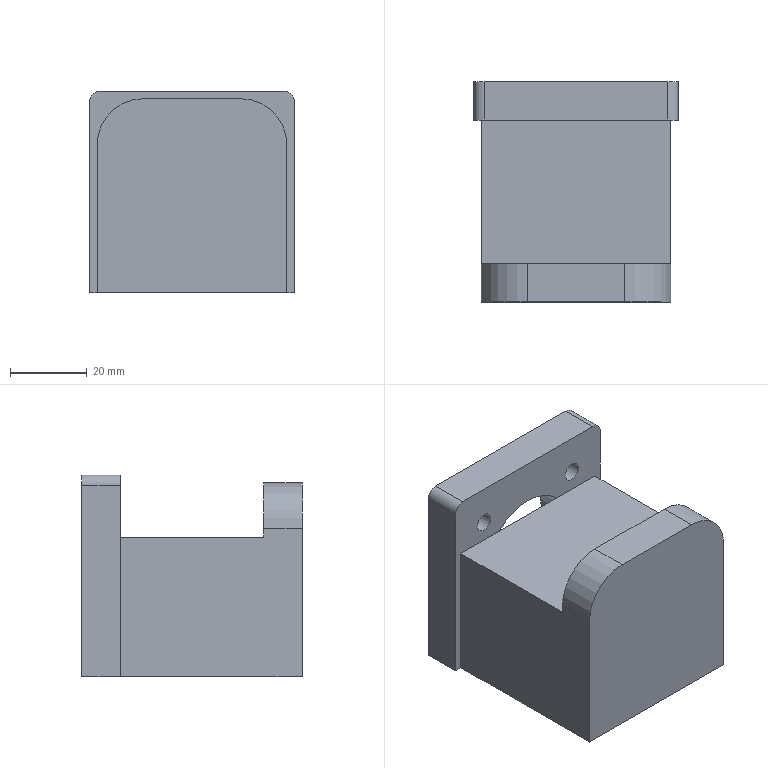Component | SolidWorks | 3359524133GTH5-400-BC(2)-1__GTH5.-BC_body6^3359524133GTH5-400-BC(2)-1 | 1 solid | 29 faces | box 53.5 x 57.5 x 52.7 mm | volume 112565 mm3 | plane 15 | cylinder 14 | commonest cylinder face diameters 4.917 x8 30 x2 24 x2 5.5 x2
STEP:
#1=COLOUR_RGB('',0.7922,0.8196,0.9333);
#2=FILL_AREA_STYLE_COLOUR('',#1);
#3=FILL_AREA_STYLE('',(#2));
#4=SURFACE_STYLE_FILL_AREA(#3);
#5=SURFACE_SIDE_STYLE('',(#4));
#6=SURFACE_STYLE_USAGE(.BOTH.,#5);
#7=PRESENTATION_STYLE_ASSIGNMENT((#6));
#8=CARTESIAN_POINT('',(13.795,57.972,-86.659));
#9=VERTEX_POINT('',#8);
#10=CARTESIAN_POINT('',(13.626,57.972,-87.072));
#11=VERTEX_POINT('',#10);
#12=CARTESIAN_POINT('',(14.216,57.972,-87.072));
#13=DIRECTION('',(0.,-1.,-0.));
#14=DIRECTION('',(1.,0.,0.));
#15=AXIS2_PLACEMENT_3D('',#12,#13,#14);
#16=CIRCLE('',#15,0.5906);
#17=EDGE_CURVE('',#9,#11,#16,.T.);
#18=ORIENTED_EDGE('',*,*,#17,.T.);
#19=CARTESIAN_POINT('',(13.626,58.366,-87.072));
#20=VERTEX_POINT('',#19);
#21=CARTESIAN_POINT('',(13.626,57.972,-87.072));
#22=DIRECTION('',(0.,1.,0.));
#23=VECTOR('',#22,39.37);
#24=LINE('',#21,#23);
#25=EDGE_CURVE('',#11,#20,#24,.T.);
#26=ORIENTED_EDGE('',*,*,#25,.T.);
#27=CARTESIAN_POINT('',(14.807,58.366,-87.072));
#28=VERTEX_POINT('',#27);
#29=CARTESIAN_POINT('',(14.216,58.366,-87.072));
#30=DIRECTION('',(0.,-1.,-0.));
#31=DIRECTION('',(1.,0.,0.));
#32=AXIS2_PLACEMENT_3D('',#29,#30,#31);
#33=CIRCLE('',#32,0.5906);
#34=EDGE_CURVE('',#28,#20,#33,.T.);
#35=ORIENTED_EDGE('',*,*,#34,.F.);
#36=CARTESIAN_POINT('',(14.807,57.972,-87.072));
#37=VERTEX_POINT('',#36);
#38=CARTESIAN_POINT('',(14.807,57.972,-87.072));
#39=DIRECTION('',(0.,1.,0.));
#40=VECTOR('',#39,39.37);
#41=LINE('',#38,#40);
#42=EDGE_CURVE('',#37,#28,#41,.T.);
#43=ORIENTED_EDGE('',*,*,#42,.F.);
#44=CARTESIAN_POINT('',(14.638,57.972,-86.659));
#45=VERTEX_POINT('',#44);
#46=CARTESIAN_POINT('',(14.216,57.972,-87.072));
#47=DIRECTION('',(0.,-1.,-0.));
#48=DIRECTION('',(1.,0.,0.));
#49=AXIS2_PLACEMENT_3D('',#46,#47,#48);
#50=CIRCLE('',#49,0.5906);
#51=EDGE_CURVE('',#37,#45,#50,.T.);
#52=ORIENTED_EDGE('',*,*,#51,.T.);
#53=CARTESIAN_POINT('',(14.216,57.972,-87.072));
#54=DIRECTION('',(0.,-1.,-0.));
#55=DIRECTION('',(1.,0.,0.));
#56=AXIS2_PLACEMENT_3D('',#53,#54,#55);
#57=CIRCLE('',#56,0.5906);
#58=EDGE_CURVE('',#45,#9,#57,.T.);
#59=ORIENTED_EDGE('',*,*,#58,.T.);
#60=EDGE_LOOP('',(#18,#26,#35,#43,#52,#59));
#61=FACE_OUTER_BOUND('',#60,.T.);
#62=CARTESIAN_POINT('',(14.216,57.972,-87.072));
#63=DIRECTION('',(0.,1.,0.));
#64=DIRECTION('',(1.,0.,0.));
#65=AXIS2_PLACEMENT_3D('',#62,#63,#64);
#66=CYLINDRICAL_SURFACE('',#65,0.5906);
#67=ADVANCED_FACE('',(#61),#66,.F.);
#68=CARTESIAN_POINT('',(13.673,57.972,-87.714));
#69=VERTEX_POINT('',#68);
#70=CARTESIAN_POINT('',(13.48,57.972,-87.714));
#71=VERTEX_POINT('',#70);
#72=CARTESIAN_POINT('',(13.577,57.972,-87.714));
#73=DIRECTION('',(0.,-1.,-0.));
#74=DIRECTION('',(1.,0.,0.));
#75=AXIS2_PLACEMENT_3D('',#72,#73,#74);
#76=CIRCLE('',#75,0.09679);
#77=EDGE_CURVE('',#69,#71,#76,.T.);
#78=ORIENTED_EDGE('',*,*,#77,.T.);
#79=CARTESIAN_POINT('',(13.48,58.366,-87.714));
#80=VERTEX_POINT('',#79);
#81=CARTESIAN_POINT('',(13.48,57.972,-87.714));
#82=DIRECTION('',(0.,1.,0.));
#83=VECTOR('',#82,39.37);
#84=LINE('',#81,#83);
#85=EDGE_CURVE('',#71,#80,#84,.T.);
#86=ORIENTED_EDGE('',*,*,#85,.T.);
#87=CARTESIAN_POINT('',(13.673,58.366,-87.714));
#88=VERTEX_POINT('',#87);
#89=CARTESIAN_POINT('',(13.577,58.366,-87.714));
#90=DIRECTION('',(0.,-1.,-0.));
#91=DIRECTION('',(1.,0.,0.));
#92=AXIS2_PLACEMENT_3D('',#89,#90,#91);
#93=CIRCLE('',#92,0.09679);
#94=EDGE_CURVE('',#88,#80,#93,.T.);
#95=ORIENTED_EDGE('',*,*,#94,.F.);
#96=CARTESIAN_POINT('',(13.673,57.972,-87.714));
#97=DIRECTION('',(0.,1.,0.));
#98=VECTOR('',#97,39.37);
#99=LINE('',#96,#98);
#100=EDGE_CURVE('',#69,#88,#99,.T.);
#101=ORIENTED_EDGE('',*,*,#100,.F.);
#102=EDGE_LOOP('',(#78,#86,#95,#101));
#103=FACE_OUTER_BOUND('',#102,.T.);
#104=CARTESIAN_POINT('',(13.577,57.972,-87.714));
#105=DIRECTION('',(0.,1.,0.));
#106=DIRECTION('',(1.,0.,0.));
#107=AXIS2_PLACEMENT_3D('',#104,#105,#106);
#108=CYLINDRICAL_SURFACE('',#107,0.09679);
#109=ADVANCED_FACE('',(#103),#108,.F.);
#110=CARTESIAN_POINT('',(14.953,57.972,-87.714));
#111=VERTEX_POINT('',#110);
#112=CARTESIAN_POINT('',(14.759,57.972,-87.714));
#113=VERTEX_POINT('',#112);
#114=CARTESIAN_POINT('',(14.856,57.972,-87.714));
#115=DIRECTION('',(0.,-1.,-0.));
#116=DIRECTION('',(1.,0.,0.));
#117=AXIS2_PLACEMENT_3D('',#114,#115,#116);
#118=CIRCLE('',#117,0.09679);
#119=EDGE_CURVE('',#111,#113,#118,.T.);
#120=ORIENTED_EDGE('',*,*,#119,.T.);
#121=CARTESIAN_POINT('',(14.759,58.366,-87.714));
#122=VERTEX_POINT('',#121);
#123=CARTESIAN_POINT('',(14.759,57.972,-87.714));
#124=DIRECTION('',(0.,1.,0.));
#125=VECTOR('',#124,39.37);
#126=LINE('',#123,#125);
#127=EDGE_CURVE('',#113,#122,#126,.T.);
#128=ORIENTED_EDGE('',*,*,#127,.T.);
#129=CARTESIAN_POINT('',(14.953,58.366,-87.714));
#130=VERTEX_POINT('',#129);
#131=CARTESIAN_POINT('',(14.856,58.366,-87.714));
#132=DIRECTION('',(0.,-1.,-0.));
#133=DIRECTION('',(1.,0.,0.));
#134=AXIS2_PLACEMENT_3D('',#131,#132,#133);
#135=CIRCLE('',#134,0.09679);
#136=EDGE_CURVE('',#130,#122,#135,.T.);
#137=ORIENTED_EDGE('',*,*,#136,.F.);
#138=CARTESIAN_POINT('',(14.953,57.972,-87.714));
#139=DIRECTION('',(0.,1.,0.));
#140=VECTOR('',#139,39.37);
#141=LINE('',#138,#140);
#142=EDGE_CURVE('',#111,#130,#141,.T.);
#143=ORIENTED_EDGE('',*,*,#142,.F.);
#144=EDGE_LOOP('',(#120,#128,#137,#143));
#145=FACE_OUTER_BOUND('',#144,.T.);
#146=CARTESIAN_POINT('',(14.856,57.972,-87.714));
#147=DIRECTION('',(0.,1.,0.));
#148=DIRECTION('',(1.,0.,0.));
#149=AXIS2_PLACEMENT_3D('',#146,#147,#148);
#150=CYLINDRICAL_SURFACE('',#149,0.09679);
#151=ADVANCED_FACE('',(#145),#150,.F.);
#152=CARTESIAN_POINT('',(13.673,57.972,-86.434));
#153=VERTEX_POINT('',#152);
#154=CARTESIAN_POINT('',(13.48,57.972,-86.434));
#155=VERTEX_POINT('',#154);
#156=CARTESIAN_POINT('',(13.577,57.972,-86.434));
#157=DIRECTION('',(0.,-1.,-0.));
#158=DIRECTION('',(1.,0.,0.));
#159=AXIS2_PLACEMENT_3D('',#156,#157,#158);
#160=CIRCLE('',#159,0.09679);
#161=EDGE_CURVE('',#153,#155,#160,.T.);
#162=ORIENTED_EDGE('',*,*,#161,.T.);
#163=CARTESIAN_POINT('',(13.48,58.366,-86.434));
#164=VERTEX_POINT('',#163);
#165=CARTESIAN_POINT('',(13.48,57.972,-86.434));
#166=DIRECTION('',(0.,1.,0.));
#167=VECTOR('',#166,39.37);
#168=LINE('',#165,#167);
#169=EDGE_CURVE('',#155,#164,#168,.T.);
#170=ORIENTED_EDGE('',*,*,#169,.T.);
#171=CARTESIAN_POINT('',(13.673,58.366,-86.434));
#172=VERTEX_POINT('',#171);
#173=CARTESIAN_POINT('',(13.577,58.366,-86.434));
#174=DIRECTION('',(0.,-1.,-0.));
#175=DIRECTION('',(1.,0.,0.));
#176=AXIS2_PLACEMENT_3D('',#173,#174,#175);
#177=CIRCLE('',#176,0.09679);
#178=EDGE_CURVE('',#172,#164,#177,.T.);
#179=ORIENTED_EDGE('',*,*,#178,.F.);
#180=CARTESIAN_POINT('',(13.673,57.972,-86.434));
#181=DIRECTION('',(0.,1.,0.));
#182=VECTOR('',#181,39.37);
#183=LINE('',#180,#182);
#184=EDGE_CURVE('',#153,#172,#183,.T.);
#185=ORIENTED_EDGE('',*,*,#184,.F.);
#186=EDGE_LOOP('',(#162,#170,#179,#185));
#187=FACE_OUTER_BOUND('',#186,.T.);
#188=CARTESIAN_POINT('',(13.577,57.972,-86.434));
#189=DIRECTION('',(0.,1.,0.));
#190=DIRECTION('',(1.,0.,0.));
#191=AXIS2_PLACEMENT_3D('',#188,#189,#190);
#192=CYLINDRICAL_SURFACE('',#191,0.09679);
#193=ADVANCED_FACE('',(#187),#192,.F.);
#194=CARTESIAN_POINT('',(14.953,57.972,-86.434));
#195=VERTEX_POINT('',#194);
#196=CARTESIAN_POINT('',(14.759,57.972,-86.434));
#197=VERTEX_POINT('',#196);
#198=CARTESIAN_POINT('',(14.856,57.972,-86.434));
#199=DIRECTION('',(0.,-1.,-0.));
#200=DIRECTION('',(1.,0.,0.));
#201=AXIS2_PLACEMENT_3D('',#198,#199,#200);
#202=CIRCLE('',#201,0.09679);
#203=EDGE_CURVE('',#195,#197,#202,.T.);
#204=ORIENTED_EDGE('',*,*,#203,.T.);
#205=CARTESIAN_POINT('',(14.759,58.366,-86.434));
#206=VERTEX_POINT('',#205);
#207=CARTESIAN_POINT('',(14.759,57.972,-86.434));
#208=DIRECTION('',(0.,1.,0.));
#209=VECTOR('',#208,39.37);
#210=LINE('',#207,#209);
#211=EDGE_CURVE('',#197,#206,#210,.T.);
#212=ORIENTED_EDGE('',*,*,#211,.T.);
#213=CARTESIAN_POINT('',(14.953,58.366,-86.434));
#214=VERTEX_POINT('',#213);
#215=CARTESIAN_POINT('',(14.856,58.366,-86.434));
#216=DIRECTION('',(0.,-1.,-0.));
#217=DIRECTION('',(1.,0.,0.));
#218=AXIS2_PLACEMENT_3D('',#215,#216,#217);
#219=CIRCLE('',#218,0.09679);
#220=EDGE_CURVE('',#214,#206,#219,.T.);
#221=ORIENTED_EDGE('',*,*,#220,.F.);
#222=CARTESIAN_POINT('',(14.953,57.972,-86.434));
#223=DIRECTION('',(0.,1.,0.));
#224=VECTOR('',#223,39.37);
#225=LINE('',#222,#224);
#226=EDGE_CURVE('',#195,#214,#225,.T.);
#227=ORIENTED_EDGE('',*,*,#226,.F.);
#228=EDGE_LOOP('',(#204,#212,#221,#227));
#229=FACE_OUTER_BOUND('',#228,.T.);
#230=CARTESIAN_POINT('',(14.856,57.972,-86.434));
#231=DIRECTION('',(0.,1.,0.));
#232=DIRECTION('',(1.,0.,0.));
#233=AXIS2_PLACEMENT_3D('',#230,#231,#232);
#234=CYLINDRICAL_SURFACE('',#233,0.09679);
#235=ADVANCED_FACE('',(#229),#234,.F.);
#236=ORIENTED_EDGE('',*,*,#211,.F.);
#237=CARTESIAN_POINT('',(14.856,57.972,-86.434));
#238=DIRECTION('',(0.,-1.,-0.));
#239=DIRECTION('',(1.,0.,0.));
#240=AXIS2_PLACEMENT_3D('',#237,#238,#239);
#241=CIRCLE('',#240,0.09679);
#242=EDGE_CURVE('',#197,#195,#241,.T.);
#243=ORIENTED_EDGE('',*,*,#242,.T.);
#244=ORIENTED_EDGE('',*,*,#226,.T.);
#245=CARTESIAN_POINT('',(14.856,58.366,-86.434));
#246=DIRECTION('',(0.,-1.,-0.));
#247=DIRECTION('',(1.,0.,0.));
#248=AXIS2_PLACEMENT_3D('',#245,#246,#247);
#249=CIRCLE('',#248,0.09679);
#250=EDGE_CURVE('',#206,#214,#249,.T.);
#251=ORIENTED_EDGE('',*,*,#250,.F.);
#252=EDGE_LOOP('',(#236,#243,#244,#251));
#253=FACE_OUTER_BOUND('',#252,.T.);
#254=CARTESIAN_POINT('',(14.856,57.972,-86.434));
#255=DIRECTION('',(0.,1.,0.));
#256=DIRECTION('',(1.,0.,0.));
#257=AXIS2_PLACEMENT_3D('',#254,#255,#256);
#258=CYLINDRICAL_SURFACE('',#257,0.09679);
#259=ADVANCED_FACE('',(#253),#258,.F.);
#260=ORIENTED_EDGE('',*,*,#169,.F.);
#261=CARTESIAN_POINT('',(13.577,57.972,-86.434));
#262=DIRECTION('',(0.,-1.,-0.));
#263=DIRECTION('',(1.,0.,0.));
#264=AXIS2_PLACEMENT_3D('',#261,#262,#263);
#265=CIRCLE('',#264,0.09679);
#266=EDGE_CURVE('',#155,#153,#265,.T.);
#267=ORIENTED_EDGE('',*,*,#266,.T.);
#268=ORIENTED_EDGE('',*,*,#184,.T.);
#269=CARTESIAN_POINT('',(13.577,58.366,-86.434));
#270=DIRECTION('',(0.,-1.,-0.));
#271=DIRECTION('',(1.,0.,0.));
#272=AXIS2_PLACEMENT_3D('',#269,#270,#271);
#273=CIRCLE('',#272,0.09679);
#274=EDGE_CURVE('',#164,#172,#273,.T.);
#275=ORIENTED_EDGE('',*,*,#274,.F.);
#276=EDGE_LOOP('',(#260,#267,#268,#275));
#277=FACE_OUTER_BOUND('',#276,.T.);
#278=CARTESIAN_POINT('',(13.577,57.972,-86.434));
#279=DIRECTION('',(0.,1.,0.));
#280=DIRECTION('',(1.,0.,0.));
#281=AXIS2_PLACEMENT_3D('',#278,#279,#280);
#282=CYLINDRICAL_SURFACE('',#281,0.09679);
#283=ADVANCED_FACE('',(#277),#282,.F.);
#284=ORIENTED_EDGE('',*,*,#119,.F.);
#285=CARTESIAN_POINT('',(14.856,57.972,-87.714));
#286=DIRECTION('',(0.,-1.,-0.));
#287=DIRECTION('',(1.,0.,0.));
#288=AXIS2_PLACEMENT_3D('',#285,#286,#287);
#289=CIRCLE('',#288,0.09679);
#290=EDGE_CURVE('',#113,#111,#289,.T.);
#291=ORIENTED_EDGE('',*,*,#290,.F.);
#292=EDGE_LOOP('',(#284,#291));
#293=FACE_OUTER_BOUND('',#292,.T.);
#294=CARTESIAN_POINT('',(14.856,57.972,-87.617));
#295=DIRECTION('',(0.,1.,0.));
#296=DIRECTION('',(-1.,0.,0.));
#297=AXIS2_PLACEMENT_3D('',#294,#295,#296);
#298=PLANE('',#297);
#299=ADVANCED_FACE('',(#293),#298,.T.);
#300=ORIENTED_EDGE('',*,*,#127,.F.);
#301=ORIENTED_EDGE('',*,*,#290,.T.);
#302=ORIENTED_EDGE('',*,*,#142,.T.);
#303=CARTESIAN_POINT('',(14.856,58.366,-87.714));
#304=DIRECTION('',(0.,-1.,-0.));
#305=DIRECTION('',(1.,0.,0.));
#306=AXIS2_PLACEMENT_3D('',#303,#304,#305);
#307=CIRCLE('',#306,0.09679);
#308=EDGE_CURVE('',#122,#130,#307,.T.);
#309=ORIENTED_EDGE('',*,*,#308,.F.);
#310=EDGE_LOOP('',(#300,#301,#302,#309));
#311=FACE_OUTER_BOUND('',#310,.T.);
#312=CARTESIAN_POINT('',(14.856,57.972,-87.714));
#313=DIRECTION('',(0.,1.,0.));
#314=DIRECTION('',(1.,0.,0.));
#315=AXIS2_PLACEMENT_3D('',#312,#313,#314);
#316=CYLINDRICAL_SURFACE('',#315,0.09679);
#317=ADVANCED_FACE('',(#311),#316,.F.);
#318=ORIENTED_EDGE('',*,*,#77,.F.);
#319=CARTESIAN_POINT('',(13.577,57.972,-87.714));
#320=DIRECTION('',(0.,-1.,-0.));
#321=DIRECTION('',(1.,0.,0.));
#322=AXIS2_PLACEMENT_3D('',#319,#320,#321);
#323=CIRCLE('',#322,0.09679);
#324=EDGE_CURVE('',#71,#69,#323,.T.);
#325=ORIENTED_EDGE('',*,*,#324,.F.);
#326=EDGE_LOOP('',(#318,#325));
#327=FACE_OUTER_BOUND('',#326,.T.);
#328=CARTESIAN_POINT('',(13.577,57.972,-87.617));
#329=DIRECTION('',(0.,1.,0.));
#330=DIRECTION('',(-1.,0.,0.));
#331=AXIS2_PLACEMENT_3D('',#328,#329,#330);
#332=PLANE('',#331);
#333=ADVANCED_FACE('',(#327),#332,.T.);
#334=ORIENTED_EDGE('',*,*,#85,.F.);
#335=ORIENTED_EDGE('',*,*,#324,.T.);
#336=ORIENTED_EDGE('',*,*,#100,.T.);
#337=CARTESIAN_POINT('',(13.577,58.366,-87.714));
#338=DIRECTION('',(0.,-1.,-0.));
#339=DIRECTION('',(1.,0.,0.));
#340=AXIS2_PLACEMENT_3D('',#337,#338,#339);
#341=CIRCLE('',#340,0.09679);
#342=EDGE_CURVE('',#80,#88,#341,.T.);
#343=ORIENTED_EDGE('',*,*,#342,.F.);
#344=EDGE_LOOP('',(#334,#335,#336,#343));
#345=FACE_OUTER_BOUND('',#344,.T.);
#346=CARTESIAN_POINT('',(13.577,57.972,-87.714));
#347=DIRECTION('',(0.,1.,0.));
#348=DIRECTION('',(1.,0.,0.));
#349=AXIS2_PLACEMENT_3D('',#346,#347,#348);
#350=CYLINDRICAL_SURFACE('',#349,0.09679);
#351=ADVANCED_FACE('',(#345),#350,.F.);
#352=ORIENTED_EDGE('',*,*,#17,.F.);
#353=CARTESIAN_POINT('',(13.242,57.972,-86.659));
#354=DIRECTION('',(1.,0.,0.));
#355=VECTOR('',#354,39.37);
#356=LINE('',#353,#355);
#357=EDGE_CURVE('',#9,#45,#356,.T.);
#358=ORIENTED_EDGE('',*,*,#357,.T.);
#359=ORIENTED_EDGE('',*,*,#51,.F.);
#360=CARTESIAN_POINT('',(14.216,57.972,-87.072));
#361=DIRECTION('',(0.,-1.,-0.));
#362=DIRECTION('',(1.,0.,0.));
#363=AXIS2_PLACEMENT_3D('',#360,#361,#362);
#364=CIRCLE('',#363,0.5906);
#365=EDGE_CURVE('',#11,#37,#364,.T.);
#366=ORIENTED_EDGE('',*,*,#365,.F.);
#367=EDGE_LOOP('',(#352,#358,#359,#366));
#368=FACE_OUTER_BOUND('',#367,.T.);
#369=CARTESIAN_POINT('',(14.216,57.972,-86.482));
#370=DIRECTION('',(0.,1.,0.));
#371=DIRECTION('',(-1.,0.,0.));
#372=AXIS2_PLACEMENT_3D('',#369,#370,#371);
#373=PLANE('',#372);
#374=ADVANCED_FACE('',(#368),#373,.T.);
#375=ORIENTED_EDGE('',*,*,#25,.F.);
#376=ORIENTED_EDGE('',*,*,#365,.T.);
#377=ORIENTED_EDGE('',*,*,#42,.T.);
#378=CARTESIAN_POINT('',(14.216,58.366,-87.072));
#379=DIRECTION('',(0.,-1.,-0.));
#380=DIRECTION('',(1.,0.,0.));
#381=AXIS2_PLACEMENT_3D('',#378,#379,#380);
#382=CIRCLE('',#381,0.5906);
#383=EDGE_CURVE('',#20,#28,#382,.T.);
#384=ORIENTED_EDGE('',*,*,#383,.F.);
#385=EDGE_LOOP('',(#375,#376,#377,#384));
#386=FACE_OUTER_BOUND('',#385,.T.);
#387=CARTESIAN_POINT('',(14.216,57.972,-87.072));
#388=DIRECTION('',(0.,1.,0.));
#389=DIRECTION('',(1.,0.,0.));
#390=AXIS2_PLACEMENT_3D('',#387,#388,#389);
#391=CYLINDRICAL_SURFACE('',#390,0.5906);
#392=ADVANCED_FACE('',(#386),#391,.F.);
#393=CARTESIAN_POINT('',(13.242,57.972,-86.659));
#394=VERTEX_POINT('',#393);
#395=CARTESIAN_POINT('',(13.242,57.972,-86.659));
#396=DIRECTION('',(1.,0.,0.));
#397=VECTOR('',#396,39.37);
#398=LINE('',#395,#397);
#399=EDGE_CURVE('',#394,#9,#398,.T.);
#400=ORIENTED_EDGE('',*,*,#399,.F.);
#401=CARTESIAN_POINT('',(13.242,56.496,-86.659));
#402=VERTEX_POINT('',#401);
#403=CARTESIAN_POINT('',(13.242,56.496,-86.659));
#404=DIRECTION('',(0.,1.,0.));
#405=VECTOR('',#404,39.37);
#406=LINE('',#403,#405);
#407=EDGE_CURVE('',#402,#394,#406,.T.);
#408=ORIENTED_EDGE('',*,*,#407,.F.);
#409=CARTESIAN_POINT('',(15.191,56.496,-86.659));
#410=VERTEX_POINT('',#409);
#411=CARTESIAN_POINT('',(13.242,56.496,-86.659));
#412=DIRECTION('',(1.,0.,0.));
#413=VECTOR('',#412,39.37);
#414=LINE('',#411,#413);
#415=EDGE_CURVE('',#402,#410,#414,.T.);
#416=ORIENTED_EDGE('',*,*,#415,.T.);
#417=CARTESIAN_POINT('',(15.191,57.972,-86.659));
#418=VERTEX_POINT('',#417);
#419=CARTESIAN_POINT('',(15.191,56.496,-86.659));
#420=DIRECTION('',(0.,1.,0.));
#421=VECTOR('',#420,39.37);
#422=LINE('',#419,#421);
#423=EDGE_CURVE('',#410,#418,#422,.T.);
#424=ORIENTED_EDGE('',*,*,#423,.T.);
#425=CARTESIAN_POINT('',(13.242,57.972,-86.659));
#426=DIRECTION('',(1.,0.,0.));
#427=VECTOR('',#426,39.37);
#428=LINE('',#425,#427);
#429=EDGE_CURVE('',#45,#418,#428,.T.);
#430=ORIENTED_EDGE('',*,*,#429,.F.);
#431=ORIENTED_EDGE('',*,*,#357,.F.);
#432=EDGE_LOOP('',(#400,#408,#416,#424,#430,#431));
#433=FACE_OUTER_BOUND('',#432,.T.);
#434=CARTESIAN_POINT('',(13.242,56.496,-86.659));
#435=DIRECTION('',(0.,-0.,1.));
#436=DIRECTION('',(0.,-1.,-0.));
#437=AXIS2_PLACEMENT_3D('',#434,#435,#436);
#438=PLANE('',#437);
#439=ADVANCED_FACE('',(#433),#438,.T.);
#440=CARTESIAN_POINT('',(14.718,56.496,-86.1));
#441=VERTEX_POINT('',#440);
#442=CARTESIAN_POINT('',(13.714,56.496,-86.1));
#443=VERTEX_POINT('',#442);
#444=CARTESIAN_POINT('',(14.718,56.496,-86.1));
#445=DIRECTION('',(-1.,0.,0.));
#446=VECTOR('',#445,39.37);
#447=LINE('',#444,#446);
#448=EDGE_CURVE('',#441,#443,#447,.T.);
#449=ORIENTED_EDGE('',*,*,#448,.F.);
#450=CARTESIAN_POINT('',(15.191,56.496,-86.572));
#451=VERTEX_POINT('',#450);
#452=CARTESIAN_POINT('',(14.718,56.496,-86.572));
#453=DIRECTION('',(0.,-1.,-0.));
#454=DIRECTION('',(1.,0.,0.));
#455=AXIS2_PLACEMENT_3D('',#452,#453,#454);
#456=CIRCLE('',#455,0.4724);
#457=EDGE_CURVE('',#451,#441,#456,.T.);
#458=ORIENTED_EDGE('',*,*,#457,.F.);
#459=CARTESIAN_POINT('',(15.191,56.496,-86.659));
#460=DIRECTION('',(0.,0.,1.));
#461=VECTOR('',#460,39.37);
#462=LINE('',#459,#461);
#463=EDGE_CURVE('',#410,#451,#462,.T.);
#464=ORIENTED_EDGE('',*,*,#463,.F.);
#465=ORIENTED_EDGE('',*,*,#415,.F.);
#466=CARTESIAN_POINT('',(13.242,56.496,-86.572));
#467=VERTEX_POINT('',#466);
#468=CARTESIAN_POINT('',(13.242,56.496,-86.068));
#469=DIRECTION('',(0.,-0.,-1.));
#470=VECTOR('',#469,39.37);
#471=LINE('',#468,#470);
#472=EDGE_CURVE('',#467,#402,#471,.T.);
#473=ORIENTED_EDGE('',*,*,#472,.F.);
#474=CARTESIAN_POINT('',(13.714,56.496,-86.572));
#475=DIRECTION('',(0.,-1.,-0.));
#476=DIRECTION('',(1.,0.,0.));
#477=AXIS2_PLACEMENT_3D('',#474,#475,#476);
#478=CIRCLE('',#477,0.4724);
#479=EDGE_CURVE('',#443,#467,#478,.T.);
#480=ORIENTED_EDGE('',*,*,#479,.F.);
#481=EDGE_LOOP('',(#449,#458,#464,#465,#473,#480));
#482=FACE_OUTER_BOUND('',#481,.T.);
#483=CARTESIAN_POINT('',(14.216,56.496,-88.163));
#484=DIRECTION('',(0.,-1.,0.));
#485=DIRECTION('',(0.,0.,1.));
#486=AXIS2_PLACEMENT_3D('',#483,#484,#485);
#487=PLANE('',#486);
#488=ADVANCED_FACE('',(#482),#487,.F.);
#489=ORIENTED_EDGE('',*,*,#161,.F.);
#490=ORIENTED_EDGE('',*,*,#266,.F.);
#491=EDGE_LOOP('',(#489,#490));
#492=FACE_BOUND('',#491,.T.);
#493=ORIENTED_EDGE('',*,*,#203,.F.);
#494=ORIENTED_EDGE('',*,*,#242,.F.);
#495=EDGE_LOOP('',(#493,#494));
#496=FACE_BOUND('',#495,.T.);
#497=ORIENTED_EDGE('',*,*,#399,.T.);
#498=ORIENTED_EDGE('',*,*,#58,.F.);
#499=ORIENTED_EDGE('',*,*,#429,.T.);
#500=CARTESIAN_POINT('',(15.191,57.972,-88.096));
#501=VERTEX_POINT('',#500);
#502=CARTESIAN_POINT('',(15.191,57.972,-88.096));
#503=DIRECTION('',(0.,0.,1.));
#504=VECTOR('',#503,39.37);
#505=LINE('',#502,#504);
#506=EDGE_CURVE('',#501,#418,#505,.T.);
#507=ORIENTED_EDGE('',*,*,#506,.F.);
#508=CARTESIAN_POINT('',(15.27,57.972,-88.096));
#509=VERTEX_POINT('',#508);
#510=CARTESIAN_POINT('',(13.163,57.972,-88.096));
#511=DIRECTION('',(-1.,0.,0.));
#512=VECTOR('',#511,39.37);
#513=LINE('',#510,#512);
#514=EDGE_CURVE('',#509,#501,#513,.T.);
#515=ORIENTED_EDGE('',*,*,#514,.F.);
#516=CARTESIAN_POINT('',(15.27,57.972,-86.129));
#517=VERTEX_POINT('',#516);
#518=CARTESIAN_POINT('',(15.27,57.972,-88.096));
#519=DIRECTION('',(0.,-0.,-1.));
#520=VECTOR('',#519,39.37);
#521=LINE('',#518,#520);
#522=EDGE_CURVE('',#517,#509,#521,.T.);
#523=ORIENTED_EDGE('',*,*,#522,.F.);
#524=CARTESIAN_POINT('',(15.161,57.972,-86.021));
#525=VERTEX_POINT('',#524);
#526=CARTESIAN_POINT('',(15.161,57.972,-86.129));
#527=DIRECTION('',(0.,1.,0.));
#528=DIRECTION('',(1.,0.,0.));
#529=AXIS2_PLACEMENT_3D('',#526,#527,#528);
#530=CIRCLE('',#529,0.1083);
#531=EDGE_CURVE('',#525,#517,#530,.T.);
#532=ORIENTED_EDGE('',*,*,#531,.F.);
#533=CARTESIAN_POINT('',(13.272,57.972,-86.021));
#534=VERTEX_POINT('',#533);
#535=CARTESIAN_POINT('',(15.161,57.972,-86.021));
#536=DIRECTION('',(1.,0.,0.));
#537=VECTOR('',#536,39.37);
#538=LINE('',#535,#537);
#539=EDGE_CURVE('',#534,#525,#538,.T.);
#540=ORIENTED_EDGE('',*,*,#539,.F.);
#541=CARTESIAN_POINT('',(13.163,57.972,-86.129));
#542=VERTEX_POINT('',#541);
#543=CARTESIAN_POINT('',(13.272,57.972,-86.129));
#544=DIRECTION('',(0.,1.,0.));
#545=DIRECTION('',(1.,0.,0.));
#546=AXIS2_PLACEMENT_3D('',#543,#544,#545);
#547=CIRCLE('',#546,0.1083);
#548=EDGE_CURVE('',#542,#534,#547,.T.);
#549=ORIENTED_EDGE('',*,*,#548,.F.);
#550=CARTESIAN_POINT('',(13.163,57.972,-88.096));
#551=VERTEX_POINT('',#550);
#552=CARTESIAN_POINT('',(13.163,57.972,-86.129));
#553=DIRECTION('',(0.,0.,1.));
#554=VECTOR('',#553,39.37);
#555=LINE('',#552,#554);
#556=EDGE_CURVE('',#551,#542,#555,.T.);
#557=ORIENTED_EDGE('',*,*,#556,.F.);
#558=CARTESIAN_POINT('',(13.242,57.972,-88.096));
#559=VERTEX_POINT('',#558);
#560=CARTESIAN_POINT('',(13.163,57.972,-88.096));
#561=DIRECTION('',(-1.,0.,0.));
#562=VECTOR('',#561,39.37);
#563=LINE('',#560,#562);
#564=EDGE_CURVE('',#559,#551,#563,.T.);
#565=ORIENTED_EDGE('',*,*,#564,.F.);
#566=CARTESIAN_POINT('',(13.242,57.972,-86.572));
#567=DIRECTION('',(0.,-0.,-1.));
#568=VECTOR('',#567,39.37);
#569=LINE('',#566,#568);
#570=EDGE_CURVE('',#394,#559,#569,.T.);
#571=ORIENTED_EDGE('',*,*,#570,.F.);
#572=EDGE_LOOP('',(#497,#498,#499,#507,#515,#523,#532,#540,#549,#557,#565,#571));
#573=FACE_OUTER_BOUND('',#572,.T.);
#574=CARTESIAN_POINT('',(14.216,57.972,-88.163));
#575=DIRECTION('',(0.,-1.,0.));
#576=DIRECTION('',(0.,0.,1.));
#577=AXIS2_PLACEMENT_3D('',#574,#575,#576);
#578=PLANE('',#577);
#579=ADVANCED_FACE('',(#492,#496,#573),#578,.T.);
#580=CARTESIAN_POINT('',(15.191,56.102,-86.572));
#581=VERTEX_POINT('',#580);
#582=CARTESIAN_POINT('',(15.191,55.709,-86.572));
#583=DIRECTION('',(0.,1.,0.));
#584=VECTOR('',#583,39.37);
#585=LINE('',#582,#584);
#586=EDGE_CURVE('',#581,#451,#585,.T.);
#587=ORIENTED_EDGE('',*,*,#586,.T.);
#588=ORIENTED_EDGE('',*,*,#457,.T.);
#589=CARTESIAN_POINT('',(14.718,56.102,-86.1));
#590=VERTEX_POINT('',#589);
#591=CARTESIAN_POINT('',(14.718,55.709,-86.1));
#592=DIRECTION('',(0.,1.,0.));
#593=VECTOR('',#592,39.37);
#594=LINE('',#591,#593);
#595=EDGE_CURVE('',#590,#441,#594,.T.);
#596=ORIENTED_EDGE('',*,*,#595,.F.);
#597=CARTESIAN_POINT('',(14.718,56.102,-86.572));
#598=DIRECTION('',(0.,1.,0.));
#599=DIRECTION('',(1.,0.,0.));
#600=AXIS2_PLACEMENT_3D('',#597,#598,#599);
#601=CIRCLE('',#600,0.4724);
#602=EDGE_CURVE('',#590,#581,#601,.T.);
#603=ORIENTED_EDGE('',*,*,#602,.T.);
#604=EDGE_LOOP('',(#587,#588,#596,#603));
#605=FACE_OUTER_BOUND('',#604,.T.);
#606=CARTESIAN_POINT('',(14.718,55.709,-86.572));
#607=DIRECTION('',(0.,-1.,-0.));
#608=DIRECTION('',(-1.,0.,0.));
#609=AXIS2_PLACEMENT_3D('',#606,#607,#608);
#610=CYLINDRICAL_SURFACE('',#609,0.4724);
#611=ADVANCED_FACE('',(#605),#610,.T.);
#612=ORIENTED_EDGE('',*,*,#595,.T.);
#613=ORIENTED_EDGE('',*,*,#448,.T.);
#614=CARTESIAN_POINT('',(13.714,56.102,-86.1));
#615=VERTEX_POINT('',#614);
#616=CARTESIAN_POINT('',(13.714,55.709,-86.1));
#617=DIRECTION('',(0.,1.,0.));
#618=VECTOR('',#617,39.37);
#619=LINE('',#616,#618);
#620=EDGE_CURVE('',#615,#443,#619,.T.);
#621=ORIENTED_EDGE('',*,*,#620,.F.);
#622=CARTESIAN_POINT('',(13.272,56.102,-86.1));
#623=DIRECTION('',(1.,0.,0.));
#624=VECTOR('',#623,39.37);
#625=LINE('',#622,#624);
#626=EDGE_CURVE('',#615,#590,#625,.T.);
#627=ORIENTED_EDGE('',*,*,#626,.T.);
#628=EDGE_LOOP('',(#612,#613,#621,#627));
#629=FACE_OUTER_BOUND('',#628,.T.);
#630=CARTESIAN_POINT('',(14.718,55.709,-86.1));
#631=DIRECTION('',(0.,-0.,-1.));
#632=DIRECTION('',(1.,0.,0.));
#633=AXIS2_PLACEMENT_3D('',#630,#631,#632);
#634=PLANE('',#633);
#635=ADVANCED_FACE('',(#629),#634,.F.);
#636=ORIENTED_EDGE('',*,*,#620,.T.);
#637=ORIENTED_EDGE('',*,*,#479,.T.);
#638=CARTESIAN_POINT('',(13.242,56.102,-86.572));
#639=VERTEX_POINT('',#638);
#640=CARTESIAN_POINT('',(13.242,55.709,-86.572));
#641=DIRECTION('',(0.,1.,0.));
#642=VECTOR('',#641,39.37);
#643=LINE('',#640,#642);
#644=EDGE_CURVE('',#639,#467,#643,.T.);
#645=ORIENTED_EDGE('',*,*,#644,.F.);
#646=CARTESIAN_POINT('',(13.714,56.102,-86.572));
#647=DIRECTION('',(0.,1.,0.));
#648=DIRECTION('',(1.,0.,0.));
#649=AXIS2_PLACEMENT_3D('',#646,#647,#648);
#650=CIRCLE('',#649,0.4724);
#651=EDGE_CURVE('',#639,#615,#650,.T.);
#652=ORIENTED_EDGE('',*,*,#651,.T.);
#653=EDGE_LOOP('',(#636,#637,#645,#652));
#654=FACE_OUTER_BOUND('',#653,.T.);
#655=CARTESIAN_POINT('',(13.714,55.709,-86.572));
#656=DIRECTION('',(0.,-1.,-0.));
#657=DIRECTION('',(-1.,0.,0.));
#658=AXIS2_PLACEMENT_3D('',#655,#656,#657);
#659=CYLINDRICAL_SURFACE('',#658,0.4724);
#660=ADVANCED_FACE('',(#654),#659,.T.);
#661=CARTESIAN_POINT('',(15.191,56.102,-88.096));
#662=VERTEX_POINT('',#661);
#663=CARTESIAN_POINT('',(15.191,55.709,-88.096));
#664=DIRECTION('',(0.,1.,0.));
#665=VECTOR('',#664,39.37);
#666=LINE('',#663,#665);
#667=EDGE_CURVE('',#662,#501,#666,.T.);
#668=ORIENTED_EDGE('',*,*,#667,.F.);
#669=CARTESIAN_POINT('',(13.242,56.102,-88.096));
#670=VERTEX_POINT('',#669);
#671=CARTESIAN_POINT('',(13.163,56.102,-88.096));
#672=DIRECTION('',(1.,-0.,-0.));
#673=VECTOR('',#672,39.37);
#674=LINE('',#671,#673);
#675=EDGE_CURVE('',#670,#662,#674,.T.);
#676=ORIENTED_EDGE('',*,*,#675,.F.);
#677=CARTESIAN_POINT('',(13.242,55.709,-88.096));
#678=DIRECTION('',(0.,1.,0.));
#679=VECTOR('',#678,39.37);
#680=LINE('',#677,#679);
#681=EDGE_CURVE('',#670,#559,#680,.T.);
#682=ORIENTED_EDGE('',*,*,#681,.T.);
#683=ORIENTED_EDGE('',*,*,#564,.T.);
#684=CARTESIAN_POINT('',(13.163,58.366,-88.096));
#685=VERTEX_POINT('',#684);
#686=CARTESIAN_POINT('',(13.163,58.366,-88.096));
#687=DIRECTION('',(0.,-1.,-0.));
#688=VECTOR('',#687,39.37);
#689=LINE('',#686,#688);
#690=EDGE_CURVE('',#685,#551,#689,.T.);
#691=ORIENTED_EDGE('',*,*,#690,.F.);
#692=CARTESIAN_POINT('',(15.27,58.366,-88.096));
#693=VERTEX_POINT('',#692);
#694=CARTESIAN_POINT('',(13.163,58.366,-88.096));
#695=DIRECTION('',(1.,-0.,-0.));
#696=VECTOR('',#695,39.37);
#697=LINE('',#694,#696);
#698=EDGE_CURVE('',#685,#693,#697,.T.);
#699=ORIENTED_EDGE('',*,*,#698,.T.);
#700=CARTESIAN_POINT('',(15.27,58.366,-88.096));
#701=DIRECTION('',(0.,-1.,-0.));
#702=VECTOR('',#701,39.37);
#703=LINE('',#700,#702);
#704=EDGE_CURVE('',#693,#509,#703,.T.);
#705=ORIENTED_EDGE('',*,*,#704,.T.);
#706=ORIENTED_EDGE('',*,*,#514,.T.);
#707=EDGE_LOOP('',(#668,#676,#682,#683,#691,#699,#705,#706));
#708=FACE_OUTER_BOUND('',#707,.T.);
#709=CARTESIAN_POINT('',(13.163,58.366,-88.096));
#710=DIRECTION('',(-0.,0.,-1.));
#711=DIRECTION('',(0.,1.,0.));
#712=AXIS2_PLACEMENT_3D('',#709,#710,#711);
#713=PLANE('',#712);
#714=ADVANCED_FACE('',(#708),#713,.T.);
#715=CARTESIAN_POINT('',(15.161,58.366,-86.021));
#716=VERTEX_POINT('',#715);
#717=CARTESIAN_POINT('',(15.161,58.366,-86.021));
#718=DIRECTION('',(0.,-1.,-0.));
#719=VECTOR('',#718,39.37);
#720=LINE('',#717,#719);
#721=EDGE_CURVE('',#716,#525,#720,.T.);
#722=ORIENTED_EDGE('',*,*,#721,.T.);
#723=ORIENTED_EDGE('',*,*,#531,.T.);
#724=CARTESIAN_POINT('',(15.27,58.366,-86.129));
#725=VERTEX_POINT('',#724);
#726=CARTESIAN_POINT('',(15.27,58.366,-86.129));
#727=DIRECTION('',(0.,-1.,-0.));
#728=VECTOR('',#727,39.37);
#729=LINE('',#726,#728);
#730=EDGE_CURVE('',#725,#517,#729,.T.);
#731=ORIENTED_EDGE('',*,*,#730,.F.);
#732=CARTESIAN_POINT('',(15.161,58.366,-86.129));
#733=DIRECTION('',(0.,-1.,-0.));
#734=DIRECTION('',(1.,0.,0.));
#735=AXIS2_PLACEMENT_3D('',#732,#733,#734);
#736=CIRCLE('',#735,0.1083);
#737=EDGE_CURVE('',#725,#716,#736,.T.);
#738=ORIENTED_EDGE('',*,*,#737,.T.);
#739=EDGE_LOOP('',(#722,#723,#731,#738));
#740=FACE_OUTER_BOUND('',#739,.T.);
#741=CARTESIAN_POINT('',(15.161,58.366,-86.129));
#742=DIRECTION('',(0.,1.,0.));
#743=DIRECTION('',(1.,0.,0.));
#744=AXIS2_PLACEMENT_3D('',#741,#742,#743);
#745=CYLINDRICAL_SURFACE('',#744,0.1083);
#746=ADVANCED_FACE('',(#740),#745,.T.);
#747=CARTESIAN_POINT('',(13.272,58.366,-86.021));
#748=VERTEX_POINT('',#747);
#749=CARTESIAN_POINT('',(13.272,58.366,-86.021));
#750=DIRECTION('',(0.,-1.,-0.));
#751=VECTOR('',#750,39.37);
#752=LINE('',#749,#751);
#753=EDGE_CURVE('',#748,#534,#752,.T.);
#754=ORIENTED_EDGE('',*,*,#753,.T.);
#755=ORIENTED_EDGE('',*,*,#539,.T.);
#756=ORIENTED_EDGE('',*,*,#721,.F.);
#757=CARTESIAN_POINT('',(15.161,58.366,-86.021));
#758=DIRECTION('',(-1.,0.,0.));
#759=VECTOR('',#758,39.37);
#760=LINE('',#757,#759);
#761=EDGE_CURVE('',#716,#748,#760,.T.);
#762=ORIENTED_EDGE('',*,*,#761,.T.);
#763=EDGE_LOOP('',(#754,#755,#756,#762));
#764=FACE_OUTER_BOUND('',#763,.T.);
#765=CARTESIAN_POINT('',(15.161,58.366,-86.021));
#766=DIRECTION('',(0.,-0.,1.));
#767=DIRECTION('',(0.,-1.,-0.));
#768=AXIS2_PLACEMENT_3D('',#765,#766,#767);
#769=PLANE('',#768);
#770=ADVANCED_FACE('',(#764),#769,.T.);
#771=CARTESIAN_POINT('',(15.191,56.102,-86.129));
#772=DIRECTION('',(0.,-0.,-1.));
#773=VECTOR('',#772,39.37);
#774=LINE('',#771,#773);
#775=EDGE_CURVE('',#581,#662,#774,.T.);
#776=ORIENTED_EDGE('',*,*,#775,.F.);
#777=ORIENTED_EDGE('',*,*,#602,.F.);
#778=ORIENTED_EDGE('',*,*,#626,.F.);
#779=ORIENTED_EDGE('',*,*,#651,.F.);
#780=CARTESIAN_POINT('',(13.242,56.102,-86.129));
#781=DIRECTION('',(0.,0.,1.));
#782=VECTOR('',#781,39.37);
#783=LINE('',#780,#782);
#784=EDGE_CURVE('',#670,#639,#783,.T.);
#785=ORIENTED_EDGE('',*,*,#784,.F.);
#786=ORIENTED_EDGE('',*,*,#675,.T.);
#787=EDGE_LOOP('',(#776,#777,#778,#779,#785,#786));
#788=FACE_OUTER_BOUND('',#787,.T.);
#789=CARTESIAN_POINT('',(13.272,56.102,-86.129));
#790=DIRECTION('',(0.,-1.,0.));
#791=DIRECTION('',(0.,0.,1.));
#792=AXIS2_PLACEMENT_3D('',#789,#790,#791);
#793=PLANE('',#792);
#794=ADVANCED_FACE('',(#788),#793,.T.);
#795=ORIENTED_EDGE('',*,*,#34,.T.);
#796=ORIENTED_EDGE('',*,*,#383,.T.);
#797=EDGE_LOOP('',(#795,#796));
#798=FACE_BOUND('',#797,.T.);
#799=ORIENTED_EDGE('',*,*,#94,.T.);
#800=ORIENTED_EDGE('',*,*,#342,.T.);
#801=EDGE_LOOP('',(#799,#800));
#802=FACE_BOUND('',#801,.T.);
#803=ORIENTED_EDGE('',*,*,#136,.T.);
#804=ORIENTED_EDGE('',*,*,#308,.T.);
#805=EDGE_LOOP('',(#803,#804));
#806=FACE_BOUND('',#805,.T.);
#807=ORIENTED_EDGE('',*,*,#178,.T.);
#808=ORIENTED_EDGE('',*,*,#274,.T.);
#809=EDGE_LOOP('',(#807,#808));
#810=FACE_BOUND('',#809,.T.);
#811=ORIENTED_EDGE('',*,*,#220,.T.);
#812=ORIENTED_EDGE('',*,*,#250,.T.);
#813=EDGE_LOOP('',(#811,#812));
#814=FACE_BOUND('',#813,.T.);
#815=CARTESIAN_POINT('',(13.163,58.366,-86.129));
#816=VERTEX_POINT('',#815);
#817=CARTESIAN_POINT('',(13.272,58.366,-86.129));
#818=DIRECTION('',(0.,-1.,-0.));
#819=DIRECTION('',(1.,0.,0.));
#820=AXIS2_PLACEMENT_3D('',#817,#818,#819);
#821=CIRCLE('',#820,0.1083);
#822=EDGE_CURVE('',#748,#816,#821,.T.);
#823=ORIENTED_EDGE('',*,*,#822,.F.);
#824=ORIENTED_EDGE('',*,*,#761,.F.);
#825=ORIENTED_EDGE('',*,*,#737,.F.);
#826=CARTESIAN_POINT('',(15.27,58.366,-88.096));
#827=DIRECTION('',(0.,0.,1.));
#828=VECTOR('',#827,39.37);
#829=LINE('',#826,#828);
#830=EDGE_CURVE('',#693,#725,#829,.T.);
#831=ORIENTED_EDGE('',*,*,#830,.F.);
#832=ORIENTED_EDGE('',*,*,#698,.F.);
#833=CARTESIAN_POINT('',(13.163,58.366,-86.129));
#834=DIRECTION('',(0.,-0.,-1.));
#835=VECTOR('',#834,39.37);
#836=LINE('',#833,#835);
#837=EDGE_CURVE('',#816,#685,#836,.T.);
#838=ORIENTED_EDGE('',*,*,#837,.F.);
#839=EDGE_LOOP('',(#823,#824,#825,#831,#832,#838));
#840=FACE_OUTER_BOUND('',#839,.T.);
#841=CARTESIAN_POINT('',(13.272,58.366,-86.129));
#842=DIRECTION('',(0.,-1.,0.));
#843=DIRECTION('',(0.,0.,1.));
#844=AXIS2_PLACEMENT_3D('',#841,#842,#843);
#845=PLANE('',#844);
#846=ADVANCED_FACE('',(#798,#802,#806,#810,#814,#840),#845,.F.);
#847=ORIENTED_EDGE('',*,*,#407,.T.);
#848=ORIENTED_EDGE('',*,*,#570,.T.);
#849=ORIENTED_EDGE('',*,*,#681,.F.);
#850=ORIENTED_EDGE('',*,*,#784,.T.);
#851=ORIENTED_EDGE('',*,*,#644,.T.);
#852=ORIENTED_EDGE('',*,*,#472,.T.);
#853=EDGE_LOOP('',(#847,#848,#849,#850,#851,#852));
#854=FACE_OUTER_BOUND('',#853,.T.);
#855=CARTESIAN_POINT('',(13.242,55.709,-86.572));
#856=DIRECTION('',(1.,0.,0.));
#857=DIRECTION('',(0.,-0.,-1.));
#858=AXIS2_PLACEMENT_3D('',#855,#856,#857);
#859=PLANE('',#858);
#860=ADVANCED_FACE('',(#854),#859,.F.);
#861=ORIENTED_EDGE('',*,*,#423,.F.);
#862=ORIENTED_EDGE('',*,*,#463,.T.);
#863=ORIENTED_EDGE('',*,*,#586,.F.);
#864=ORIENTED_EDGE('',*,*,#775,.T.);
#865=ORIENTED_EDGE('',*,*,#667,.T.);
#866=ORIENTED_EDGE('',*,*,#506,.T.);
#867=EDGE_LOOP('',(#861,#862,#863,#864,#865,#866));
#868=FACE_OUTER_BOUND('',#867,.T.);
#869=CARTESIAN_POINT('',(15.191,55.709,-88.096));
#870=DIRECTION('',(-1.,0.,0.));
#871=DIRECTION('',(0.,-1.,-0.));
#872=AXIS2_PLACEMENT_3D('',#869,#870,#871);
#873=PLANE('',#872);
#874=ADVANCED_FACE('',(#868),#873,.F.);
#875=CARTESIAN_POINT('',(13.163,58.366,-86.129));
#876=DIRECTION('',(0.,-1.,-0.));
#877=VECTOR('',#876,39.37);
#878=LINE('',#875,#877);
#879=EDGE_CURVE('',#816,#542,#878,.T.);
#880=ORIENTED_EDGE('',*,*,#879,.T.);
#881=ORIENTED_EDGE('',*,*,#548,.T.);
#882=ORIENTED_EDGE('',*,*,#753,.F.);
#883=ORIENTED_EDGE('',*,*,#822,.T.);
#884=EDGE_LOOP('',(#880,#881,#882,#883));
#885=FACE_OUTER_BOUND('',#884,.T.);
#886=CARTESIAN_POINT('',(13.272,58.366,-86.129));
#887=DIRECTION('',(0.,1.,0.));
#888=DIRECTION('',(1.,0.,0.));
#889=AXIS2_PLACEMENT_3D('',#886,#887,#888);
#890=CYLINDRICAL_SURFACE('',#889,0.1083);
#891=ADVANCED_FACE('',(#885),#890,.T.);
#892=ORIENTED_EDGE('',*,*,#730,.T.);
#893=ORIENTED_EDGE('',*,*,#522,.T.);
#894=ORIENTED_EDGE('',*,*,#704,.F.);
#895=ORIENTED_EDGE('',*,*,#830,.T.);
#896=EDGE_LOOP('',(#892,#893,#894,#895));
#897=FACE_OUTER_BOUND('',#896,.T.);
#898=CARTESIAN_POINT('',(15.27,58.366,-88.096));
#899=DIRECTION('',(1.,0.,0.));
#900=DIRECTION('',(0.,-0.,-1.));
#901=AXIS2_PLACEMENT_3D('',#898,#899,#900);
#902=PLANE('',#901);
#903=ADVANCED_FACE('',(#897),#902,.T.);
#904=ORIENTED_EDGE('',*,*,#690,.T.);
#905=ORIENTED_EDGE('',*,*,#556,.T.);
#906=ORIENTED_EDGE('',*,*,#879,.F.);
#907=ORIENTED_EDGE('',*,*,#837,.T.);
#908=EDGE_LOOP('',(#904,#905,#906,#907));
#909=FACE_OUTER_BOUND('',#908,.T.);
#910=CARTESIAN_POINT('',(13.163,58.366,-86.129));
#911=DIRECTION('',(-1.,0.,0.));
#912=DIRECTION('',(0.,-1.,-0.));
#913=AXIS2_PLACEMENT_3D('',#910,#911,#912);
#914=PLANE('',#913);
#915=ADVANCED_FACE('',(#909),#914,.T.);
#916=CLOSED_SHELL('',(#67,#109,#151,#193,#235,#259,#283,#299,#317,#333,#351,#374,#392,#439,#488,#579,#611,#635,#660,#714,#746,#770,#794,#846,#860,#874,#891,#903,#915));
#917=MANIFOLD_SOLID_BREP('',#916);
#918=STYLED_ITEM('',(#7),#917);
#919=(LENGTH_UNIT()NAMED_UNIT(*)SI_UNIT($,.METRE.));
#920=LENGTH_MEASURE_WITH_UNIT(LENGTH_MEASURE(0.0254),#919);
#921=DIMENSIONAL_EXPONENTS(1.,0.,0.,0.,0.,0.,0.);
#922=(CONVERSION_BASED_UNIT('',#920)LENGTH_UNIT()NAMED_UNIT(#921));
#923=UNCERTAINTY_MEASURE_WITH_UNIT(LENGTH_MEASURE(0.00001),#922,'','');
#924=(NAMED_UNIT(*)PLANE_ANGLE_UNIT()SI_UNIT($,.RADIAN.));
#925=(NAMED_UNIT(*)SI_UNIT($,.STERADIAN.)SOLID_ANGLE_UNIT());
#926=(GEOMETRIC_REPRESENTATION_CONTEXT(3)GLOBAL_UNCERTAINTY_ASSIGNED_CONTEXT((#923))GLOBAL_UNIT_ASSIGNED_CONTEXT((#922,#924,#925))REPRESENTATION_CONTEXT('',''));
#927=MECHANICAL_DESIGN_GEOMETRIC_PRESENTATION_REPRESENTATION('',(#918),#926);
#928=CARTESIAN_POINT('',(0.,0.,0.));
#929=DIRECTION('',(0.,0.,1.));
#930=DIRECTION('',(1.,0.,0.));
#931=AXIS2_PLACEMENT_3D('',#928,#929,#930);
#932=(LENGTH_UNIT()NAMED_UNIT(*)SI_UNIT($,.METRE.));
#933=LENGTH_MEASURE_WITH_UNIT(LENGTH_MEASURE(0.0254),#932);
#934=DIMENSIONAL_EXPONENTS(1.,0.,0.,0.,0.,0.,0.);
#935=(CONVERSION_BASED_UNIT('',#933)LENGTH_UNIT()NAMED_UNIT(#934));
#936=UNCERTAINTY_MEASURE_WITH_UNIT(LENGTH_MEASURE(0.00001),#935,'','');
#937=(NAMED_UNIT(*)PLANE_ANGLE_UNIT()SI_UNIT($,.RADIAN.));
#938=(NAMED_UNIT(*)SI_UNIT($,.STERADIAN.)SOLID_ANGLE_UNIT());
#939=(GEOMETRIC_REPRESENTATION_CONTEXT(3)GLOBAL_UNCERTAINTY_ASSIGNED_CONTEXT((#936))GLOBAL_UNIT_ASSIGNED_CONTEXT((#935,#937,#938))REPRESENTATION_CONTEXT('',''));
#940=ADVANCED_BREP_SHAPE_REPRESENTATION('',(#917,#931),#939);
#941=PRESENTATION_LAYER_ASSIGNMENT('','',(#918));